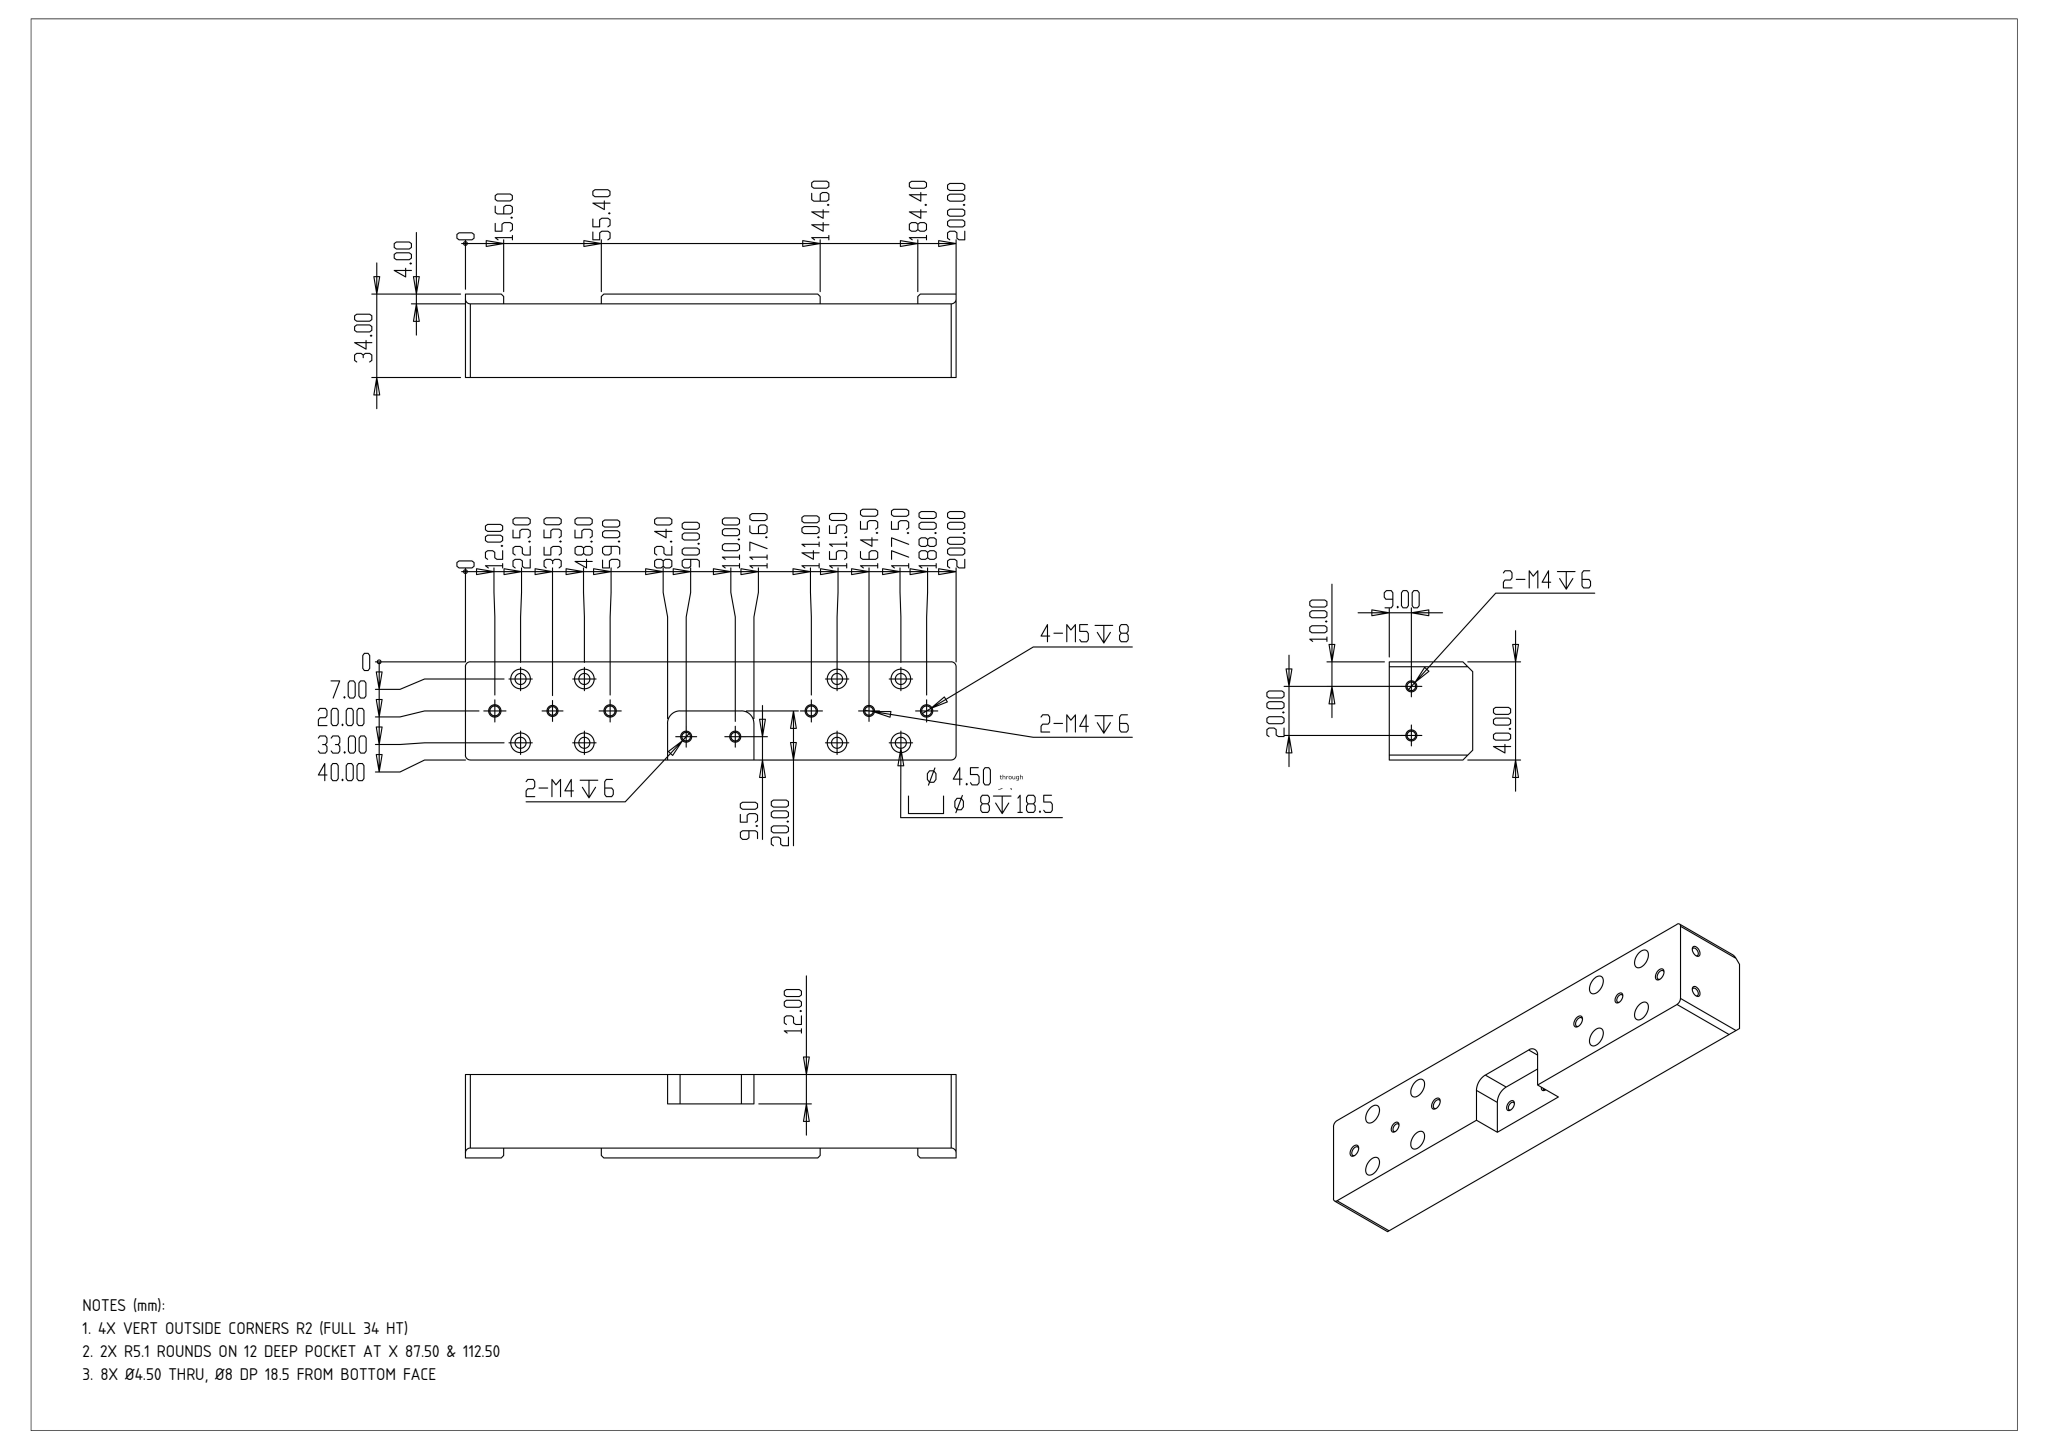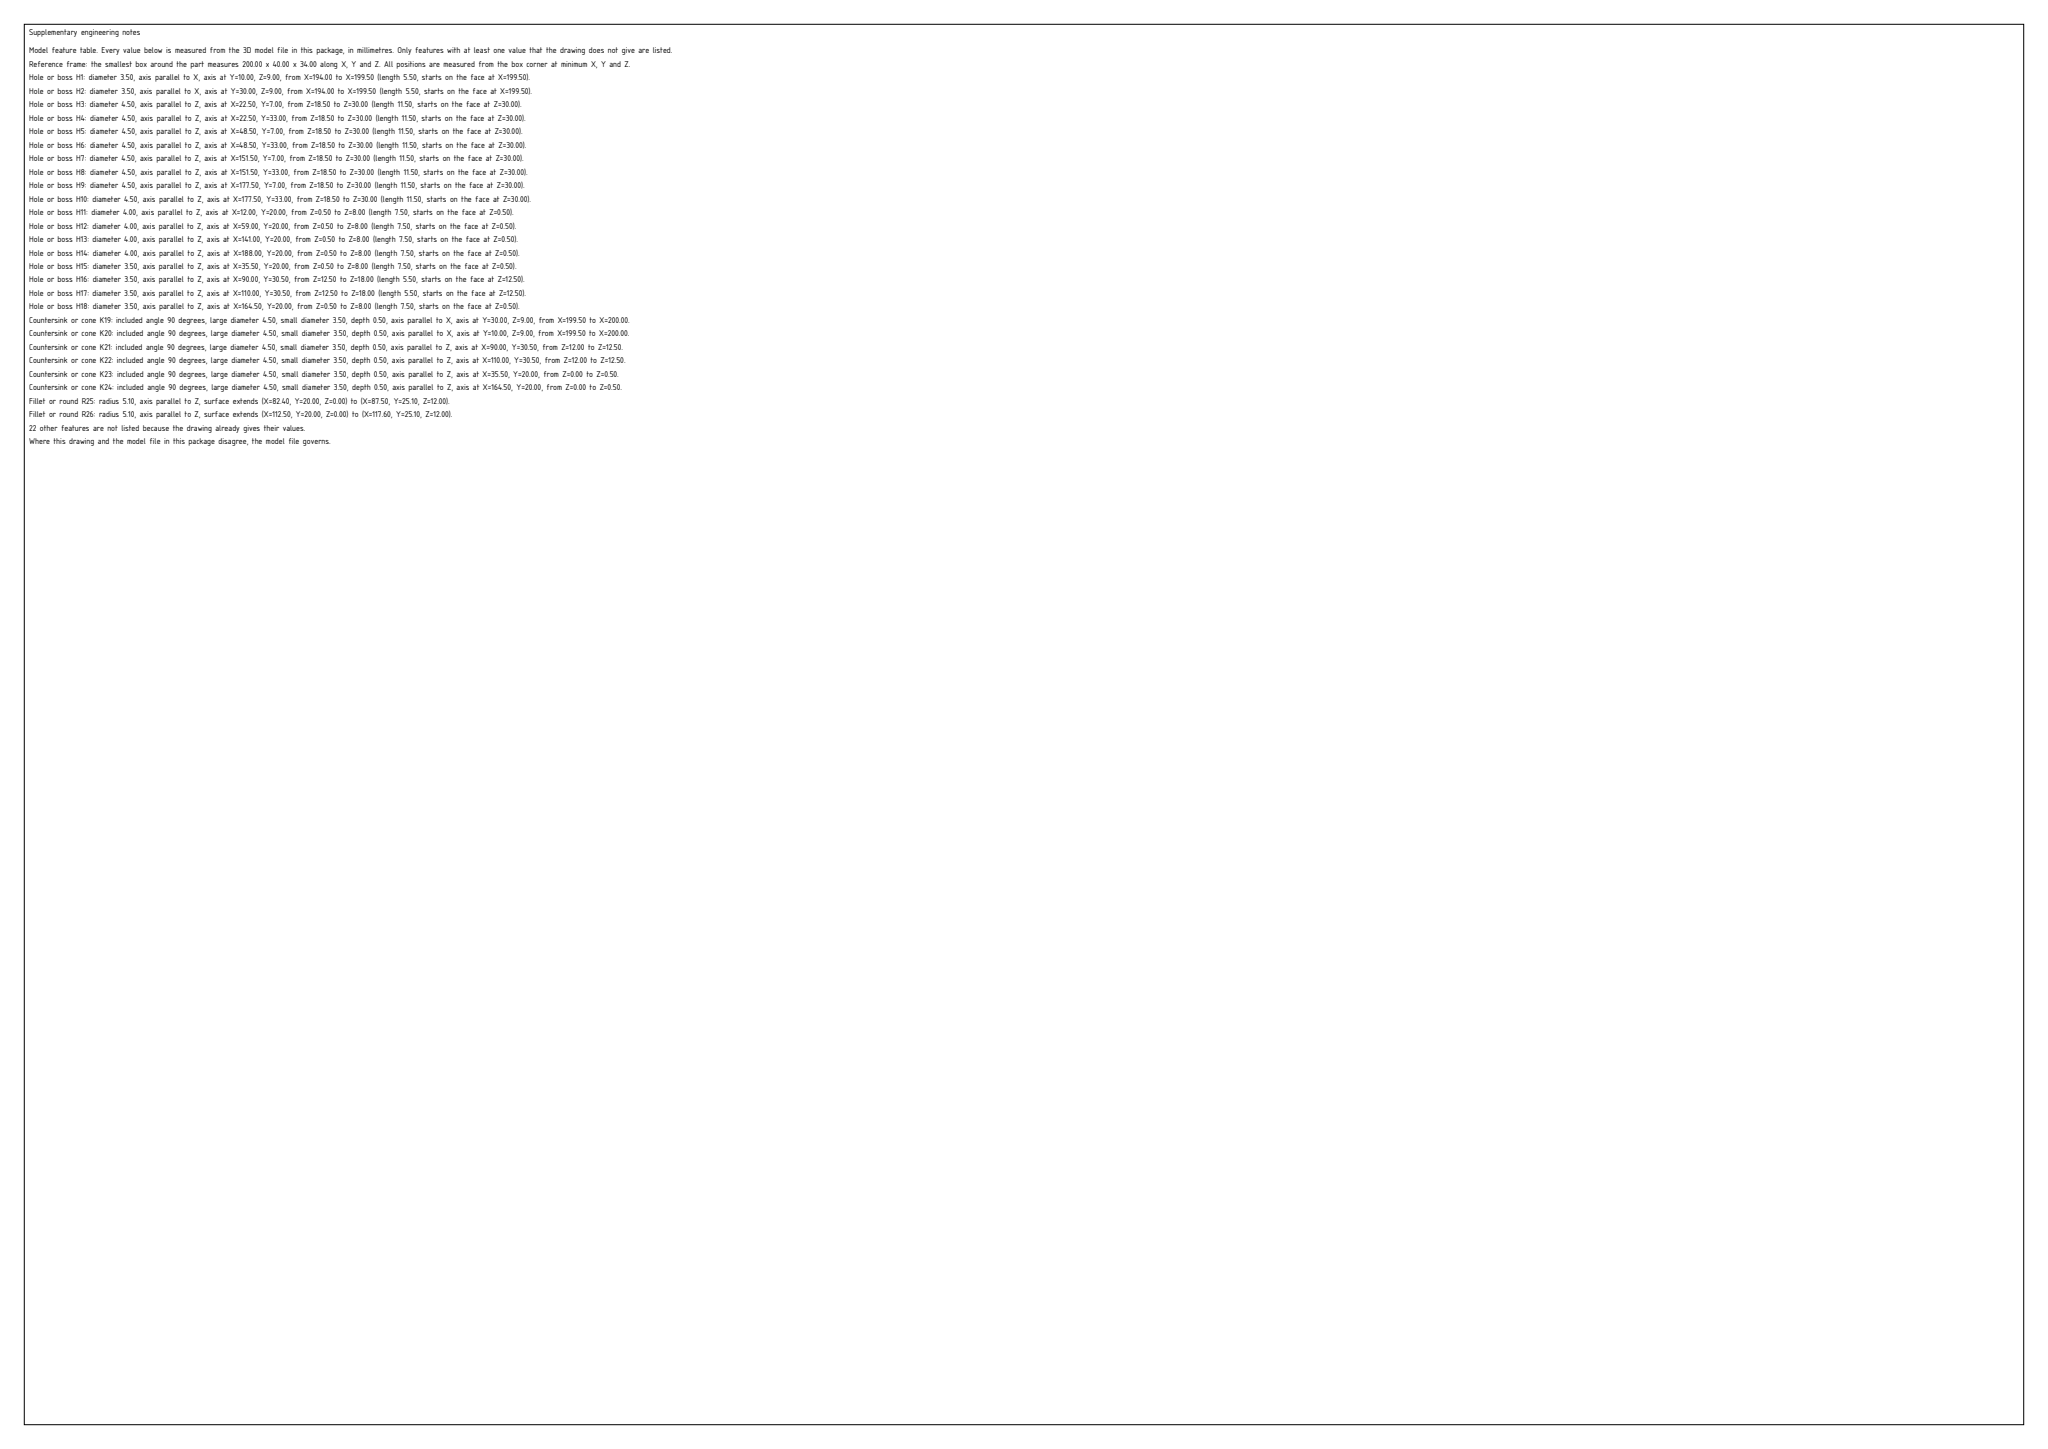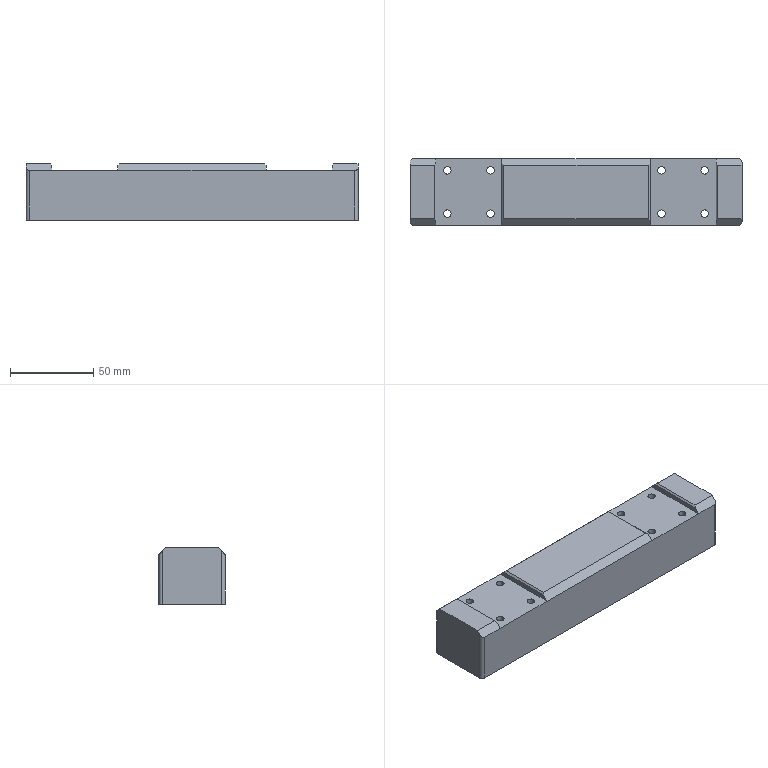Part | SolidWorks | mm | 1 solid | 124 faces | box 200 x 40 x 34 mm | volume 239148 mm3 | cylinder 58 | plane 46 | cone 20 | commonest cylinder face diameters 8 x16 4.5 x16 3.5 x12 4 x12 10.2 x2
Drawing notes:
4X VERT OUTSIDE CORNERS R2 (FULL 34 HT) | from the solid: Ø4 Z-axis cyls at (2,2),(2,38),(198,2),(198,38), L=32 -> R2 rounds
2X R5.1 ROUNDS ON 12 DEEP POCKET AT X 87.50 & 112.50 | from the solid: Ø10.2 Z-axis cyls at (87.5,25.1) & (112.5,25.1), L=12; z plane 12.0
8X Ø4.50 THRU, Ø8 DP 18.5 FROM BOTTOM FACE | from the solid: 8 Ø4.5 thru + 8 Ø8 L18.5 c'bores at x22.5/48.5/151.5/177.5, y7/33; z plane 18.5 count 8 from z=0
build123d program:
from build123d import *

# Parameters (mm, degrees)
BOSS_EXTRUDE1_DEPTH = 34
CUT_EXTRUDE1_DEPTH  = 18.5
CUT_EXTRUDE2_DEPTH  = 12
CUT_EXTRUDE3_REACH  = 145.556
CUT_EXTRUDE4_REACH  = 206.632
SKETCH6_R           = 2
SKETCH6_R_2         = 1.75
CUT_EXTRUDE5_DEPTH  = 8
SKETCH7_R           = 1.75
CUT_EXTRUDE6_DEPTH  = 6
SKETCH8_R           = 1.75
CUT_EXTRUDE7_DEPTH  = 6
CHAMFER1_SIZE       = 0.5


with BuildPart() as part:
    # Sketch1 → Boss-Extrude1 (new body)
    with BuildSketch(Plane.XY):
        with BuildLine():
            Line((-78.212, -13.199), (10.988, -13.199))
            Line((10.988, -13.199), (50.788, -13.199))
            Line((50.788, -13.199), (64.388, -13.199))
            ThreePointArc((64.388, -13.199), (65.802, -12.613), (66.388, -11.199))
            Line((66.388, -11.199), (66.388, -9.199))
            Line((66.388, -9.199), (66.388, 22.801))
            Line((66.388, 22.801), (66.388, 24.801))
            ThreePointArc((66.388, 24.801), (65.802, 26.215), (64.388, 26.801))
            Line((64.388, 26.801), (50.788, 26.801))
            Line((50.788, 26.801), (10.988, 26.801))
            Line((10.988, 26.801), (-78.212, 26.801))
            Line((-78.212, 26.801), (-118.012, 26.801))
            Line((-118.012, 26.801), (-131.612, 26.801))
            ThreePointArc((-131.612, 26.801), (-133.026, 26.215), (-133.612, 24.801))
            Line((-133.612, 24.801), (-133.612, 22.801))
            Line((-133.612, 22.801), (-133.612, -9.199))
            Line((-133.612, -9.199), (-133.612, -11.199))
            ThreePointArc((-133.612, -11.199), (-133.026, -12.613), (-131.612, -13.199))
            Line((-131.612, -13.199), (-118.012, -13.199))
            Line((-118.012, -13.199), (-78.212, -13.199))
        make_face()
        with BuildLine():
            ThreePointArc((-108.862, -6.199), (-111.112, -8.449), (-113.362, -6.199))
            ThreePointArc((-113.362, -6.199), (-111.112, -3.949), (-108.862, -6.199))
        make_face(mode=Mode.SUBTRACT)
        with BuildLine():
            ThreePointArc((-82.862, -6.199), (-85.112, -8.449), (-87.362, -6.199))
            ThreePointArc((-87.362, -6.199), (-85.112, -3.949), (-82.862, -6.199))
        make_face(mode=Mode.SUBTRACT)
        with BuildLine():
            ThreePointArc((20.138, -6.199), (17.888, -8.449), (15.638, -6.199))
            ThreePointArc((15.638, -6.199), (17.888, -3.949), (20.138, -6.199))
        make_face(mode=Mode.SUBTRACT)
        with BuildLine():
            ThreePointArc((46.138, -6.199), (43.888, -8.449), (41.638, -6.199))
            ThreePointArc((41.638, -6.199), (43.888, -3.949), (46.138, -6.199))
        make_face(mode=Mode.SUBTRACT)
        with BuildLine():
            ThreePointArc((-108.862, 19.801), (-111.112, 17.551), (-113.362, 19.801))
            ThreePointArc((-113.362, 19.801), (-111.112, 22.051), (-108.862, 19.801))
        make_face(mode=Mode.SUBTRACT)
        with BuildLine():
            ThreePointArc((-82.862, 19.801), (-85.112, 17.551), (-87.362, 19.801))
            ThreePointArc((-87.362, 19.801), (-85.112, 22.051), (-82.862, 19.801))
        make_face(mode=Mode.SUBTRACT)
        with BuildLine():
            ThreePointArc((20.138, 19.801), (17.888, 17.551), (15.638, 19.801))
            ThreePointArc((15.638, 19.801), (17.888, 22.051), (20.138, 19.801))
        make_face(mode=Mode.SUBTRACT)
        with BuildLine():
            ThreePointArc((46.138, 19.801), (43.888, 17.551), (41.638, 19.801))
            ThreePointArc((41.638, 19.801), (43.888, 22.051), (46.138, 19.801))
        make_face(mode=Mode.SUBTRACT)
    extrude(amount=BOSS_EXTRUDE1_DEPTH)

    # Sketch2 → Cut-Extrude1 (cut)
    with BuildSketch(Plane(origin=(0, 0, 0), x_dir=(-1, 0, 0), z_dir=(0, 0, -1))):
        with BuildLine():
            ThreePointArc((-21.888, 19.801), (-17.888, 15.801), (-13.888, 19.801))
            ThreePointArc((-13.888, 19.801), (-17.888, 23.801), (-21.888, 19.801))
        make_face()
        with BuildLine():
            ThreePointArc((81.112, -6.199), (85.112, -10.199), (89.112, -6.199))
            ThreePointArc((89.112, -6.199), (85.112, -2.199), (81.112, -6.199))
        make_face()
        with BuildLine():
            ThreePointArc((107.112, -6.199), (111.112, -10.199), (115.112, -6.199))
            ThreePointArc((115.112, -6.199), (111.112, -2.199), (107.112, -6.199))
        make_face()
        with BuildLine():
            ThreePointArc((-21.888, -6.199), (-17.888, -10.199), (-13.888, -6.199))
            ThreePointArc((-13.888, -6.199), (-17.888, -2.199), (-21.888, -6.199))
        make_face()
        with BuildLine():
            ThreePointArc((-47.888, 19.801), (-43.888, 15.801), (-39.888, 19.801))
            ThreePointArc((-39.888, 19.801), (-43.888, 23.801), (-47.888, 19.801))
        make_face()
        with BuildLine():
            ThreePointArc((81.112, 19.801), (85.112, 15.801), (89.112, 19.801))
            ThreePointArc((89.112, 19.801), (85.112, 23.801), (81.112, 19.801))
        make_face()
        with BuildLine():
            ThreePointArc((-47.888, -6.199), (-43.888, -10.199), (-39.888, -6.199))
            ThreePointArc((-39.888, -6.199), (-43.888, -2.199), (-47.888, -6.199))
        make_face()
        with BuildLine():
            ThreePointArc((107.112, 19.801), (111.112, 15.801), (115.112, 19.801))
            ThreePointArc((115.112, 19.801), (111.112, 23.801), (107.112, 19.801))
        make_face()
    extrude(amount=-CUT_EXTRUDE1_DEPTH, mode=Mode.SUBTRACT)

    # Sketch3 → Cut-Extrude2 (cut)
    with BuildSketch(Plane(origin=(0, 0, 0), x_dir=(-1, 0, 0), z_dir=(0, 0, -1))):
        with BuildLine():
            Line((51.212, 26.801), (51.212, 11.901))
            ThreePointArc((51.212, 11.901), (49.718, 8.295), (46.112, 6.801))
            Line((46.112, 6.801), (21.112, 6.801))
            ThreePointArc((21.112, 6.801), (17.506, 8.295), (16.012, 11.901))
            Line((16.012, 11.901), (16.012, 26.801))
            Line((16.012, 26.801), (51.212, 26.801))
        make_face()
    extrude(amount=-CUT_EXTRUDE2_DEPTH, mode=Mode.SUBTRACT)

    # Sketch4 → Cut-Extrude3 (cut, up to next)
    with BuildSketch(Plane(origin=(0, 26.801, 0), x_dir=(1, 0, 0), z_dir=(0, 1, 0)), mode=Mode.PRIVATE) as cut_extrude3_sk1:
        Polygon((50.788, -30), (50.788, -33), (51.788, -34), (9.988, -34), (10.988, -33), (10.988, -30), align=None)
    cut_extrude3_tool1 = extrude(cut_extrude3_sk1.sketch, amount=-CUT_EXTRUDE3_REACH, mode=Mode.PRIVATE) & part.part
    # Sketch4 → Cut-Extrude3 (cut, up to next)
    with BuildSketch(Plane(origin=(0, 26.801, 0), x_dir=(1, 0, 0), z_dir=(0, 1, 0)), mode=Mode.PRIVATE) as cut_extrude3_sk2:
        Polygon((-78.212, -30), (-78.212, -33), (-77.212, -34), (-119.012, -34), (-118.012, -33), (-118.012, -30), align=None)
    cut_extrude3_tool2 = extrude(cut_extrude3_sk2.sketch, amount=-CUT_EXTRUDE3_REACH, mode=Mode.PRIVATE) & part.part
    add(cut_extrude3_tool1.solids().sort_by_distance((30.888, 26.801, 32.01))[0], mode=Mode.SUBTRACT)
    add(cut_extrude3_tool2.solids().sort_by_distance((-98.112, 26.801, 32.01))[0], mode=Mode.SUBTRACT)

    # Cut-Extrude4: up to this face of the body (flat: up to its plane)
    cut_extrude4_end = Plane(part.part.faces().sort_by_distance((66.388, 6.801, 17))[0])
    # Sketch5 → Cut-Extrude4 (cut, up to the picked face)
    with BuildSketch(Plane.ZY.offset(133.612), mode=Mode.PRIVATE) as cut_extrude4_sk1:
        Polygon((34, -13.199), (34, -9.199), (30, -13.199), align=None)
    cut_extrude4_tool1 = split(extrude(cut_extrude4_sk1.sketch, amount=-CUT_EXTRUDE4_REACH, mode=Mode.PRIVATE), bisect_by=cut_extrude4_end, keep=Keep.BOTH, mode=Mode.PRIVATE)
    # Sketch5 → Cut-Extrude4 (cut, up to the picked face)
    with BuildSketch(Plane.ZY.offset(133.612), mode=Mode.PRIVATE) as cut_extrude4_sk2:
        Polygon((30, 26.801), (34, 22.801), (34, 26.801), align=None)
    cut_extrude4_tool2 = split(extrude(cut_extrude4_sk2.sketch, amount=-CUT_EXTRUDE4_REACH, mode=Mode.PRIVATE), bisect_by=cut_extrude4_end, keep=Keep.BOTH, mode=Mode.PRIVATE)
    add(cut_extrude4_tool1.solids().sort_by(Axis((-133.612, -11.866, 32.667), (1, 0, 0)))[0], mode=Mode.SUBTRACT)
    add(cut_extrude4_tool2.solids().sort_by(Axis((-133.612, 25.468, 32.667), (1, 0, 0)))[0], mode=Mode.SUBTRACT)

    # Sketch6 → Cut-Extrude5 (cut)
    with BuildSketch(Plane(origin=(0, 0, 0), x_dir=(-1, 0, 0), z_dir=(0, 0, -1))):
        with Locations((121.612, 6.801)):
            Circle(SKETCH6_R)
        with Locations((74.612, 6.801)):
            Circle(SKETCH6_R)
        with Locations((-7.388, 6.801)):
            Circle(SKETCH6_R)
        with Locations((-54.388, 6.801)):
            Circle(SKETCH6_R)
        with Locations((98.112, 6.801)):
            Circle(SKETCH6_R_2)
        with Locations((-30.888, 6.801)):
            Circle(SKETCH6_R_2)
    extrude(amount=-CUT_EXTRUDE5_DEPTH, mode=Mode.SUBTRACT)

    # Sketch7 → Cut-Extrude6 (cut)
    with BuildSketch(Plane(origin=(0, 0, 12), x_dir=(-1, 0, 0), z_dir=(0, 0, -1))):
        with Locations((43.612, 17.301)):
            Circle(SKETCH7_R)
        with Locations((23.612, 17.301)):
            Circle(SKETCH7_R)
    extrude(amount=-CUT_EXTRUDE6_DEPTH, mode=Mode.SUBTRACT)

    # Sketch8 → Cut-Extrude7 (cut)
    with BuildSketch(Plane(origin=(66.388, 0, 0), x_dir=(0, 0, -1), z_dir=(1, 0, 0))):
        with Locations((-9, 16.801)):
            Circle(SKETCH8_R)
        with Locations((-9, -3.199)):
            Circle(SKETCH8_R)
    extrude(amount=-CUT_EXTRUDE7_DEPTH, mode=Mode.SUBTRACT)

    # Chamfer1
    chamfer1_edges = [part.edges().sort_by_distance(p)[0] for p in [
        (-119.612, 6.801, 0),
        (32.638, 6.801, 0),
        (56.388, 6.801, 0),
        (9.388, 6.801, 0),
        (-72.612, 6.801, 0),
        (-96.362, 6.801, 0),
        (-41.862, 17.301, 12),
        (-21.862, 17.301, 12),
        (66.388, 16.801, 10.75),
        (66.388, -3.199, 10.75),
    ]]
    chamfer(chamfer1_edges, length=CHAMFER1_SIZE)


solid = part.part